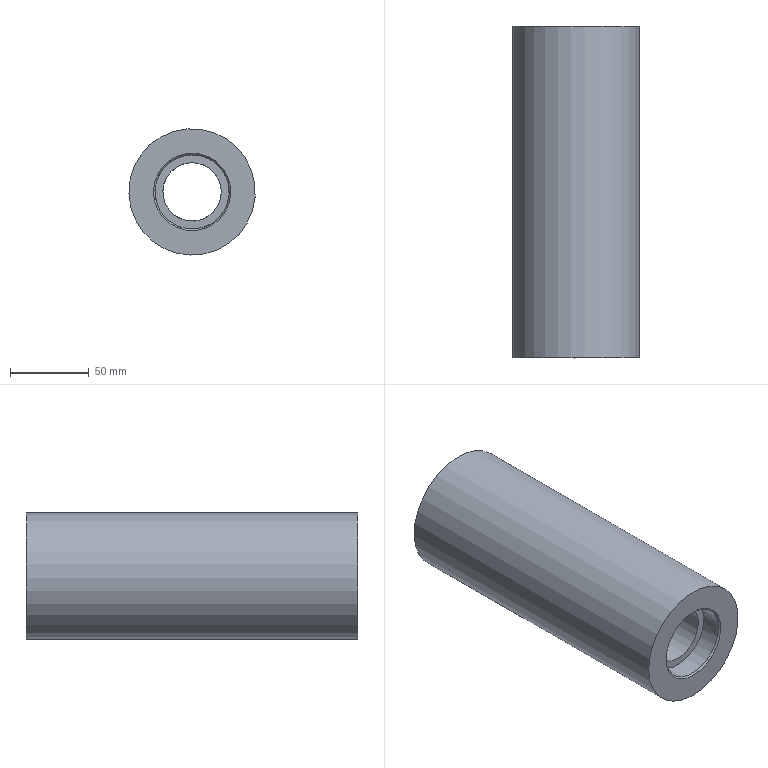Component | NX | 131_ROLLER | 1 solid | 10 faces | box 80 x 210 x 80 mm | volume 811159 mm3 | plane 4 | cylinder 4 | cone 2 | commonest cylinder face diameters 47 x2 80 x1 37 x1
STEP:
#1=CARTESIAN_POINT('',(0.,0.,0.));
#2=DIRECTION('',(0.,0.,1.));
#3=DIRECTION('',(1.,0.,0.));
#4=AXIS2_PLACEMENT_3D('',#1,#2,#3);
#5=CARTESIAN_POINT('',(613.188,-110.,-20.648));
#6=VERTEX_POINT('',#5);
#7=CARTESIAN_POINT('',(600.,-110.,0.));
#8=DIRECTION('',(-0.,1.,-0.));
#9=DIRECTION('',(0.5383,-0.,-0.8428));
#10=AXIS2_PLACEMENT_3D('',#7,#8,#9);
#11=CIRCLE('',#10,24.5);
#12=CARTESIAN_POINT('',(600.,-110.,0.));
#13=DIRECTION('',(0.,-1.,0.));
#14=DIRECTION('',(0.5383,-0.,-0.8428));
#15=AXIS2_PLACEMENT_3D('',#12,#13,#14);
#16=PLANE('',#15);
#17=CARTESIAN_POINT('',(24.5,0.));
#18=CARTESIAN_POINT('',(24.5,-42.435));
#19=CARTESIAN_POINT('',(-12.25,-21.218));
#20=CARTESIAN_POINT('',(-49.,0.));
#21=CARTESIAN_POINT('',(-12.25,21.218));
#22=CARTESIAN_POINT('',(24.5,42.435));
#23=CARTESIAN_POINT('',(24.5,0.));
#24=(BOUNDED_CURVE()B_SPLINE_CURVE(2,(#17,#18,#19,#20,#21,#22,#23),.UNSPECIFIED.,.T.,.F.)B_SPLINE_CURVE_WITH_KNOTS((1,2,2,2,2,1),(-2.094,0.,2.094,4.189,6.283,8.378),.UNSPECIFIED.)CURVE()GEOMETRIC_REPRESENTATION_ITEM()RATIONAL_B_SPLINE_CURVE((1.,0.5,1.,0.5,1.,0.5,1.))REPRESENTATION_ITEM(''));
#25=(GEOMETRIC_REPRESENTATION_CONTEXT(2)PARAMETRIC_REPRESENTATION_CONTEXT()REPRESENTATION_CONTEXT('',''));
#26=DEFINITIONAL_REPRESENTATION('',(#24),#25);
#27=PCURVE('',#16,#26);
#28=CARTESIAN_POINT('',(600.,-110.,0.));
#29=DIRECTION('',(-0.,-1.,0.));
#30=DIRECTION('',(0.5383,-0.,-0.8428));
#31=AXIS2_PLACEMENT_3D('',#28,#29,#30);
#32=CONICAL_SURFACE('',#31,24.5,0.7854);
#33=CARTESIAN_POINT('',(6.283,-0.));
#34=DIRECTION('',(-1.,0.));
#35=VECTOR('',#34,1.);
#36=LINE('',#33,#35);
#37=(GEOMETRIC_REPRESENTATION_CONTEXT(2)PARAMETRIC_REPRESENTATION_CONTEXT()REPRESENTATION_CONTEXT('',''));
#38=DEFINITIONAL_REPRESENTATION('',(#36),#37);
#39=PCURVE('',#32,#38);
#40=SURFACE_CURVE('',#11,(#27,#39),.PCURVE_S1.);
#41=EDGE_CURVE('',#6,#6,#40,.T.);
#42=ORIENTED_EDGE('',*,*,#41,.T.);
#43=EDGE_LOOP('',(#42));
#44=FACE_BOUND('',#43,.T.);
#45=CARTESIAN_POINT('',(633.711,-110.,21.531));
#46=VERTEX_POINT('',#45);
#47=CARTESIAN_POINT('',(600.,-110.,0.));
#48=DIRECTION('',(0.,-1.,0.));
#49=DIRECTION('',(0.8428,0.,0.5383));
#50=AXIS2_PLACEMENT_3D('',#47,#48,#49);
#51=CIRCLE('',#50,40.);
#52=CARTESIAN_POINT('',(-0.,0.));
#53=DIRECTION('',(0.,1.));
#54=AXIS2_PLACEMENT_2D('',#52,#53);
#55=CIRCLE('',#54,40.);
#56=(GEOMETRIC_REPRESENTATION_CONTEXT(2)PARAMETRIC_REPRESENTATION_CONTEXT()REPRESENTATION_CONTEXT('',''));
#57=DEFINITIONAL_REPRESENTATION('',(#55),#56);
#58=PCURVE('',#16,#57);
#59=CARTESIAN_POINT('',(600.,-110.,0.));
#60=DIRECTION('',(-0.,1.,-0.));
#61=DIRECTION('',(-0.5383,0.,0.8428));
#62=AXIS2_PLACEMENT_3D('',#59,#60,#61);
#63=CYLINDRICAL_SURFACE('',#62,40.);
#64=CARTESIAN_POINT('',(7.854,0.));
#65=DIRECTION('',(-1.,0.));
#66=VECTOR('',#65,1.);
#67=LINE('',#64,#66);
#68=(GEOMETRIC_REPRESENTATION_CONTEXT(2)PARAMETRIC_REPRESENTATION_CONTEXT()REPRESENTATION_CONTEXT('',''));
#69=DEFINITIONAL_REPRESENTATION('',(#67),#68);
#70=PCURVE('',#63,#69);
#71=SURFACE_CURVE('',#51,(#58,#70),.PCURVE_S1.);
#72=EDGE_CURVE('',#46,#46,#71,.T.);
#73=ORIENTED_EDGE('',*,*,#72,.T.);
#74=EDGE_LOOP('',(#73));
#75=FACE_BOUND('',#74,.T.);
#76=ADVANCED_FACE('',(#44,#75),#16,.T.);
#77=CARTESIAN_POINT('',(613.188,100.,-20.648));
#78=VERTEX_POINT('',#77);
#79=CARTESIAN_POINT('',(600.,100.,0.));
#80=DIRECTION('',(0.,-1.,0.));
#81=DIRECTION('',(0.5383,-0.,-0.8428));
#82=AXIS2_PLACEMENT_3D('',#79,#80,#81);
#83=CIRCLE('',#82,24.5);
#84=CARTESIAN_POINT('',(600.,100.,0.));
#85=DIRECTION('',(0.,-1.,0.));
#86=DIRECTION('',(0.5383,-0.,-0.8428));
#87=AXIS2_PLACEMENT_3D('',#84,#85,#86);
#88=PLANE('',#87);
#89=CARTESIAN_POINT('',(-0.,0.));
#90=DIRECTION('',(1.,0.));
#91=AXIS2_PLACEMENT_2D('',#89,#90);
#92=CIRCLE('',#91,24.5);
#93=(GEOMETRIC_REPRESENTATION_CONTEXT(2)PARAMETRIC_REPRESENTATION_CONTEXT()REPRESENTATION_CONTEXT('',''));
#94=DEFINITIONAL_REPRESENTATION('',(#92),#93);
#95=PCURVE('',#88,#94);
#96=CARTESIAN_POINT('',(600.,99.,0.));
#97=DIRECTION('',(-0.,1.,0.));
#98=DIRECTION('',(-0.5383,-0.,0.8428));
#99=AXIS2_PLACEMENT_3D('',#96,#97,#98);
#100=CONICAL_SURFACE('',#99,23.5,0.7854);
#101=CARTESIAN_POINT('',(9.425,1.));
#102=DIRECTION('',(-1.,0.));
#103=VECTOR('',#102,1.);
#104=LINE('',#101,#103);
#105=(GEOMETRIC_REPRESENTATION_CONTEXT(2)PARAMETRIC_REPRESENTATION_CONTEXT()REPRESENTATION_CONTEXT('',''));
#106=DEFINITIONAL_REPRESENTATION('',(#104),#105);
#107=PCURVE('',#100,#106);
#108=SURFACE_CURVE('',#83,(#95,#107),.PCURVE_S1.);
#109=EDGE_CURVE('',#78,#78,#108,.T.);
#110=ORIENTED_EDGE('',*,*,#109,.T.);
#111=EDGE_LOOP('',(#110));
#112=FACE_BOUND('',#111,.T.);
#113=CARTESIAN_POINT('',(633.711,100.,21.531));
#114=VERTEX_POINT('',#113);
#115=CARTESIAN_POINT('',(600.,100.,0.));
#116=DIRECTION('',(0.,-1.,0.));
#117=DIRECTION('',(0.8428,0.,0.5383));
#118=AXIS2_PLACEMENT_3D('',#115,#116,#117);
#119=CIRCLE('',#118,40.);
#120=CARTESIAN_POINT('',(-0.,0.));
#121=DIRECTION('',(0.,1.));
#122=AXIS2_PLACEMENT_2D('',#120,#121);
#123=CIRCLE('',#122,40.);
#124=(GEOMETRIC_REPRESENTATION_CONTEXT(2)PARAMETRIC_REPRESENTATION_CONTEXT()REPRESENTATION_CONTEXT('',''));
#125=DEFINITIONAL_REPRESENTATION('',(#123),#124);
#126=PCURVE('',#88,#125);
#127=CARTESIAN_POINT('',(7.854,210.));
#128=DIRECTION('',(-1.,0.));
#129=VECTOR('',#128,1.);
#130=LINE('',#127,#129);
#131=(GEOMETRIC_REPRESENTATION_CONTEXT(2)PARAMETRIC_REPRESENTATION_CONTEXT()REPRESENTATION_CONTEXT('',''));
#132=DEFINITIONAL_REPRESENTATION('',(#130),#131);
#133=PCURVE('',#63,#132);
#134=SURFACE_CURVE('',#119,(#126,#133),.PCURVE_S1.);
#135=EDGE_CURVE('',#114,#114,#134,.T.);
#136=ORIENTED_EDGE('',*,*,#135,.F.);
#137=EDGE_LOOP('',(#136));
#138=FACE_BOUND('',#137,.T.);
#139=ADVANCED_FACE('',(#112,#138),#88,.F.);
#140=ORIENTED_EDGE('',*,*,#72,.F.);
#141=CARTESIAN_POINT('',(633.711,-110.,21.531));
#142=CARTESIAN_POINT('',(633.711,100.,21.531));
#143=B_SPLINE_CURVE_WITH_KNOTS('',1,(#141,#142),.UNSPECIFIED.,.F.,.F.,(2,2),(0.,210.),.PIECEWISE_BEZIER_KNOTS.);
#144=CARTESIAN_POINT('',(7.854,0.));
#145=DIRECTION('',(0.,1.));
#146=VECTOR('',#145,1.);
#147=LINE('',#144,#146);
#148=(GEOMETRIC_REPRESENTATION_CONTEXT(2)PARAMETRIC_REPRESENTATION_CONTEXT()REPRESENTATION_CONTEXT('',''));
#149=DEFINITIONAL_REPRESENTATION('',(#147),#148);
#150=PCURVE('',#63,#149);
#151=CARTESIAN_POINT('',(1.571,0.));
#152=DIRECTION('',(0.,1.));
#153=VECTOR('',#152,1.);
#154=LINE('',#151,#153);
#155=(GEOMETRIC_REPRESENTATION_CONTEXT(2)PARAMETRIC_REPRESENTATION_CONTEXT()REPRESENTATION_CONTEXT('',''));
#156=DEFINITIONAL_REPRESENTATION('',(#154),#155);
#157=PCURVE('',#63,#156);
#158=SEAM_CURVE('',#143,(#150,#157),.PCURVE_S1.);
#159=EDGE_CURVE('',#46,#114,#158,.T.);
#160=ORIENTED_EDGE('',*,*,#159,.T.);
#161=ORIENTED_EDGE('',*,*,#135,.T.);
#162=ORIENTED_EDGE('',*,*,#159,.F.);
#163=EDGE_LOOP('',(#140,#160,#161,#162));
#164=FACE_BOUND('',#163,.T.);
#165=ADVANCED_FACE('',(#164),#63,.T.);
#166=CARTESIAN_POINT('',(619.805,99.,12.649));
#167=VERTEX_POINT('',#166);
#168=CARTESIAN_POINT('',(612.649,99.,-19.805));
#169=VERTEX_POINT('',#168);
#170=CARTESIAN_POINT('',(600.,99.,0.));
#171=DIRECTION('',(-0.,1.,0.));
#172=DIRECTION('',(0.5383,0.,-0.8428));
#173=AXIS2_PLACEMENT_3D('',#170,#171,#172);
#174=CIRCLE('',#173,23.5);
#175=CARTESIAN_POINT('',(600.,86.,0.));
#176=DIRECTION('',(-0.,1.,-0.));
#177=DIRECTION('',(-0.5383,-0.,0.8428));
#178=AXIS2_PLACEMENT_3D('',#175,#176,#177);
#179=CYLINDRICAL_SURFACE('',#178,23.5);
#180=CARTESIAN_POINT('',(-3.142,13.));
#181=DIRECTION('',(1.,0.));
#182=VECTOR('',#181,1.);
#183=LINE('',#180,#182);
#184=(GEOMETRIC_REPRESENTATION_CONTEXT(2)PARAMETRIC_REPRESENTATION_CONTEXT()REPRESENTATION_CONTEXT('',''));
#185=DEFINITIONAL_REPRESENTATION('',(#183),#184);
#186=PCURVE('',#179,#185);
#187=CARTESIAN_POINT('',(3.142,-0.));
#188=DIRECTION('',(1.,0.));
#189=VECTOR('',#188,1.);
#190=LINE('',#187,#189);
#191=(GEOMETRIC_REPRESENTATION_CONTEXT(2)PARAMETRIC_REPRESENTATION_CONTEXT()REPRESENTATION_CONTEXT('',''));
#192=DEFINITIONAL_REPRESENTATION('',(#190),#191);
#193=PCURVE('',#100,#192);
#194=SURFACE_CURVE('',#174,(#186,#193),.PCURVE_S1.);
#195=EDGE_CURVE('',#167,#169,#194,.T.);
#196=ORIENTED_EDGE('',*,*,#195,.F.);
#197=CARTESIAN_POINT('',(619.805,86.,12.649));
#198=VERTEX_POINT('',#197);
#199=CARTESIAN_POINT('',(619.805,86.,12.649));
#200=CARTESIAN_POINT('',(619.805,99.,12.649));
#201=B_SPLINE_CURVE_WITH_KNOTS('',1,(#199,#200),.UNSPECIFIED.,.F.,.F.,(2,2),(0.,13.),.PIECEWISE_BEZIER_KNOTS.);
#202=CARTESIAN_POINT('',(1.571,0.));
#203=DIRECTION('',(0.,1.));
#204=VECTOR('',#203,1.);
#205=LINE('',#202,#204);
#206=(GEOMETRIC_REPRESENTATION_CONTEXT(2)PARAMETRIC_REPRESENTATION_CONTEXT()REPRESENTATION_CONTEXT('',''));
#207=DEFINITIONAL_REPRESENTATION('',(#205),#206);
#208=PCURVE('',#179,#207);
#209=CARTESIAN_POINT('',(7.854,0.));
#210=DIRECTION('',(0.,1.));
#211=VECTOR('',#210,1.);
#212=LINE('',#209,#211);
#213=(GEOMETRIC_REPRESENTATION_CONTEXT(2)PARAMETRIC_REPRESENTATION_CONTEXT()REPRESENTATION_CONTEXT('',''));
#214=DEFINITIONAL_REPRESENTATION('',(#212),#213);
#215=PCURVE('',#179,#214);
#216=SEAM_CURVE('',#201,(#208,#215),.PCURVE_S1.);
#217=EDGE_CURVE('',#198,#167,#216,.T.);
#218=ORIENTED_EDGE('',*,*,#217,.F.);
#219=CARTESIAN_POINT('',(600.,86.,0.));
#220=DIRECTION('',(-0.,-1.,0.));
#221=DIRECTION('',(0.8428,0.,0.5383));
#222=AXIS2_PLACEMENT_3D('',#219,#220,#221);
#223=CIRCLE('',#222,23.5);
#224=CARTESIAN_POINT('',(7.854,0.));
#225=DIRECTION('',(-1.,0.));
#226=VECTOR('',#225,1.);
#227=LINE('',#224,#226);
#228=(GEOMETRIC_REPRESENTATION_CONTEXT(2)PARAMETRIC_REPRESENTATION_CONTEXT()REPRESENTATION_CONTEXT('',''));
#229=DEFINITIONAL_REPRESENTATION('',(#227),#228);
#230=PCURVE('',#179,#229);
#231=CARTESIAN_POINT('',(600.,86.,0.));
#232=DIRECTION('',(-0.,1.,-0.));
#233=DIRECTION('',(-0.5383,0.,0.8428));
#234=AXIS2_PLACEMENT_3D('',#231,#232,#233);
#235=PLANE('',#234);
#236=CARTESIAN_POINT('',(-0.,23.5));
#237=CARTESIAN_POINT('',(40.703,23.5));
#238=CARTESIAN_POINT('',(20.352,-11.75));
#239=CARTESIAN_POINT('',(-0.,-47.));
#240=CARTESIAN_POINT('',(-20.352,-11.75));
#241=CARTESIAN_POINT('',(-40.703,23.5));
#242=CARTESIAN_POINT('',(-0.,23.5));
#243=(BOUNDED_CURVE()B_SPLINE_CURVE(2,(#236,#237,#238,#239,#240,#241,#242),.UNSPECIFIED.,.T.,.F.)B_SPLINE_CURVE_WITH_KNOTS((1,2,2,2,2,1),(-2.094,0.,2.094,4.189,6.283,8.378),.UNSPECIFIED.)CURVE()GEOMETRIC_REPRESENTATION_ITEM()RATIONAL_B_SPLINE_CURVE((1.,0.5,1.,0.5,1.,0.5,1.))REPRESENTATION_ITEM(''));
#244=(GEOMETRIC_REPRESENTATION_CONTEXT(2)PARAMETRIC_REPRESENTATION_CONTEXT()REPRESENTATION_CONTEXT('',''));
#245=DEFINITIONAL_REPRESENTATION('',(#243),#244);
#246=PCURVE('',#235,#245);
#247=SURFACE_CURVE('',#223,(#230,#246),.PCURVE_S1.);
#248=EDGE_CURVE('',#198,#198,#247,.T.);
#249=ORIENTED_EDGE('',*,*,#248,.F.);
#250=ORIENTED_EDGE('',*,*,#217,.T.);
#251=CARTESIAN_POINT('',(600.,99.,0.));
#252=DIRECTION('',(-0.,1.,0.));
#253=DIRECTION('',(0.5383,0.,-0.8428));
#254=AXIS2_PLACEMENT_3D('',#251,#252,#253);
#255=CIRCLE('',#254,23.5);
#256=CARTESIAN_POINT('',(3.142,13.));
#257=DIRECTION('',(1.,0.));
#258=VECTOR('',#257,1.);
#259=LINE('',#256,#258);
#260=(GEOMETRIC_REPRESENTATION_CONTEXT(2)PARAMETRIC_REPRESENTATION_CONTEXT()REPRESENTATION_CONTEXT('',''));
#261=DEFINITIONAL_REPRESENTATION('',(#259),#260);
#262=PCURVE('',#179,#261);
#263=CARTESIAN_POINT('',(3.142,0.));
#264=DIRECTION('',(1.,-0.));
#265=VECTOR('',#264,1.);
#266=LINE('',#263,#265);
#267=(GEOMETRIC_REPRESENTATION_CONTEXT(2)PARAMETRIC_REPRESENTATION_CONTEXT()REPRESENTATION_CONTEXT('',''));
#268=DEFINITIONAL_REPRESENTATION('',(#266),#267);
#269=PCURVE('',#100,#268);
#270=SURFACE_CURVE('',#255,(#262,#269),.PCURVE_S1.);
#271=EDGE_CURVE('',#169,#167,#270,.T.);
#272=ORIENTED_EDGE('',*,*,#271,.F.);
#273=EDGE_LOOP('',(#196,#218,#249,#250,#272));
#274=FACE_BOUND('',#273,.F.);
#275=ADVANCED_FACE('',(#274),#179,.F.);
#276=CARTESIAN_POINT('',(615.591,86.,9.958));
#277=VERTEX_POINT('',#276);
#278=CARTESIAN_POINT('',(590.042,86.,15.591));
#279=VERTEX_POINT('',#278);
#280=CARTESIAN_POINT('',(600.,86.,0.));
#281=DIRECTION('',(0.,1.,-0.));
#282=DIRECTION('',(0.8428,0.,0.5383));
#283=AXIS2_PLACEMENT_3D('',#280,#281,#282);
#284=CIRCLE('',#283,18.5);
#285=CARTESIAN_POINT('',(0.,0.));
#286=DIRECTION('',(0.,1.));
#287=AXIS2_PLACEMENT_2D('',#285,#286);
#288=CIRCLE('',#287,18.5);
#289=(GEOMETRIC_REPRESENTATION_CONTEXT(2)PARAMETRIC_REPRESENTATION_CONTEXT()REPRESENTATION_CONTEXT('',''));
#290=DEFINITIONAL_REPRESENTATION('',(#288),#289);
#291=PCURVE('',#235,#290);
#292=CARTESIAN_POINT('',(600.,-114.,0.));
#293=DIRECTION('',(-0.,1.,-0.));
#294=DIRECTION('',(-0.5383,0.,0.8428));
#295=AXIS2_PLACEMENT_3D('',#292,#293,#294);
#296=CYLINDRICAL_SURFACE('',#295,18.5);
#297=CARTESIAN_POINT('',(1.571,200.));
#298=DIRECTION('',(1.,0.));
#299=VECTOR('',#298,1.);
#300=LINE('',#297,#299);
#301=(GEOMETRIC_REPRESENTATION_CONTEXT(2)PARAMETRIC_REPRESENTATION_CONTEXT()REPRESENTATION_CONTEXT('',''));
#302=DEFINITIONAL_REPRESENTATION('',(#300),#301);
#303=PCURVE('',#296,#302);
#304=SURFACE_CURVE('',#284,(#291,#303),.PCURVE_S1.);
#305=EDGE_CURVE('',#277,#279,#304,.T.);
#306=ORIENTED_EDGE('',*,*,#305,.F.);
#307=CARTESIAN_POINT('',(600.,86.,0.));
#308=DIRECTION('',(0.,1.,-0.));
#309=DIRECTION('',(0.8428,0.,0.5383));
#310=AXIS2_PLACEMENT_3D('',#307,#308,#309);
#311=CIRCLE('',#310,18.5);
#312=CARTESIAN_POINT('',(0.,0.));
#313=DIRECTION('',(0.,1.));
#314=AXIS2_PLACEMENT_2D('',#312,#313);
#315=CIRCLE('',#314,18.5);
#316=(GEOMETRIC_REPRESENTATION_CONTEXT(2)PARAMETRIC_REPRESENTATION_CONTEXT()REPRESENTATION_CONTEXT('',''));
#317=DEFINITIONAL_REPRESENTATION('',(#315),#316);
#318=PCURVE('',#235,#317);
#319=CARTESIAN_POINT('',(-4.712,200.));
#320=DIRECTION('',(1.,0.));
#321=VECTOR('',#320,1.);
#322=LINE('',#319,#321);
#323=(GEOMETRIC_REPRESENTATION_CONTEXT(2)PARAMETRIC_REPRESENTATION_CONTEXT()REPRESENTATION_CONTEXT('',''));
#324=DEFINITIONAL_REPRESENTATION('',(#322),#323);
#325=PCURVE('',#296,#324);
#326=SURFACE_CURVE('',#311,(#318,#325),.PCURVE_S1.);
#327=EDGE_CURVE('',#279,#277,#326,.T.);
#328=ORIENTED_EDGE('',*,*,#327,.F.);
#329=EDGE_LOOP('',(#306,#328));
#330=FACE_BOUND('',#329,.T.);
#331=ORIENTED_EDGE('',*,*,#248,.F.);
#332=EDGE_LOOP('',(#331));
#333=FACE_BOUND('',#332,.T.);
#334=ADVANCED_FACE('',(#330,#333),#235,.T.);
#335=ORIENTED_EDGE('',*,*,#109,.T.);
#336=CARTESIAN_POINT('',(612.649,99.,-19.805));
#337=CARTESIAN_POINT('',(613.188,100.,-20.648));
#338=B_SPLINE_CURVE_WITH_KNOTS('',1,(#336,#337),.UNSPECIFIED.,.F.,.F.,(2,2),(0.,1.414),.PIECEWISE_BEZIER_KNOTS.);
#339=CARTESIAN_POINT('',(3.142,0.));
#340=DIRECTION('',(0.,1.));
#341=VECTOR('',#340,1.);
#342=LINE('',#339,#341);
#343=(GEOMETRIC_REPRESENTATION_CONTEXT(2)PARAMETRIC_REPRESENTATION_CONTEXT()REPRESENTATION_CONTEXT('',''));
#344=DEFINITIONAL_REPRESENTATION('',(#342),#343);
#345=PCURVE('',#100,#344);
#346=CARTESIAN_POINT('',(9.425,0.));
#347=DIRECTION('',(0.,1.));
#348=VECTOR('',#347,1.);
#349=LINE('',#346,#348);
#350=(GEOMETRIC_REPRESENTATION_CONTEXT(2)PARAMETRIC_REPRESENTATION_CONTEXT()REPRESENTATION_CONTEXT('',''));
#351=DEFINITIONAL_REPRESENTATION('',(#349),#350);
#352=PCURVE('',#100,#351);
#353=SEAM_CURVE('',#338,(#345,#352),.PCURVE_S1.);
#354=EDGE_CURVE('',#169,#78,#353,.T.);
#355=ORIENTED_EDGE('',*,*,#354,.F.);
#356=ORIENTED_EDGE('',*,*,#271,.T.);
#357=ORIENTED_EDGE('',*,*,#195,.T.);
#358=ORIENTED_EDGE('',*,*,#354,.T.);
#359=EDGE_LOOP('',(#335,#355,#356,#357,#358));
#360=FACE_BOUND('',#359,.F.);
#361=ADVANCED_FACE('',(#360),#100,.F.);
#362=CARTESIAN_POINT('',(612.649,-109.,-19.805));
#363=VERTEX_POINT('',#362);
#364=CARTESIAN_POINT('',(600.,-109.,0.));
#365=DIRECTION('',(-0.,-1.,0.));
#366=DIRECTION('',(0.5383,-0.,-0.8428));
#367=AXIS2_PLACEMENT_3D('',#364,#365,#366);
#368=CIRCLE('',#367,23.5);
#369=CARTESIAN_POINT('',(600.,-96.,0.));
#370=DIRECTION('',(0.,-1.,0.));
#371=DIRECTION('',(0.5383,0.,-0.8428));
#372=AXIS2_PLACEMENT_3D('',#369,#370,#371);
#373=CYLINDRICAL_SURFACE('',#372,23.5);
#374=CARTESIAN_POINT('',(0.,13.));
#375=DIRECTION('',(1.,0.));
#376=VECTOR('',#375,1.);
#377=LINE('',#374,#376);
#378=(GEOMETRIC_REPRESENTATION_CONTEXT(2)PARAMETRIC_REPRESENTATION_CONTEXT()REPRESENTATION_CONTEXT('',''));
#379=DEFINITIONAL_REPRESENTATION('',(#377),#378);
#380=PCURVE('',#373,#379);
#381=CARTESIAN_POINT('',(0.,-1.));
#382=DIRECTION('',(1.,0.));
#383=VECTOR('',#382,1.);
#384=LINE('',#381,#383);
#385=(GEOMETRIC_REPRESENTATION_CONTEXT(2)PARAMETRIC_REPRESENTATION_CONTEXT()REPRESENTATION_CONTEXT('',''));
#386=DEFINITIONAL_REPRESENTATION('',(#384),#385);
#387=PCURVE('',#32,#386);
#388=SURFACE_CURVE('',#368,(#380,#387),.PCURVE_S1.);
#389=EDGE_CURVE('',#363,#363,#388,.T.);
#390=ORIENTED_EDGE('',*,*,#389,.F.);
#391=CARTESIAN_POINT('',(612.649,-96.,-19.805));
#392=VERTEX_POINT('',#391);
#393=CARTESIAN_POINT('',(612.649,-96.,-19.805));
#394=CARTESIAN_POINT('',(612.649,-109.,-19.805));
#395=B_SPLINE_CURVE_WITH_KNOTS('',1,(#393,#394),.UNSPECIFIED.,.F.,.F.,(2,2),(0.,13.),.PIECEWISE_BEZIER_KNOTS.);
#396=CARTESIAN_POINT('',(0.,0.));
#397=DIRECTION('',(0.,1.));
#398=VECTOR('',#397,1.);
#399=LINE('',#396,#398);
#400=(GEOMETRIC_REPRESENTATION_CONTEXT(2)PARAMETRIC_REPRESENTATION_CONTEXT()REPRESENTATION_CONTEXT('',''));
#401=DEFINITIONAL_REPRESENTATION('',(#399),#400);
#402=PCURVE('',#373,#401);
#403=CARTESIAN_POINT('',(6.283,0.));
#404=DIRECTION('',(0.,1.));
#405=VECTOR('',#404,1.);
#406=LINE('',#403,#405);
#407=(GEOMETRIC_REPRESENTATION_CONTEXT(2)PARAMETRIC_REPRESENTATION_CONTEXT()REPRESENTATION_CONTEXT('',''));
#408=DEFINITIONAL_REPRESENTATION('',(#406),#407);
#409=PCURVE('',#373,#408);
#410=SEAM_CURVE('',#395,(#402,#409),.PCURVE_S1.);
#411=EDGE_CURVE('',#392,#363,#410,.T.);
#412=ORIENTED_EDGE('',*,*,#411,.F.);
#413=CARTESIAN_POINT('',(619.805,-96.,12.649));
#414=VERTEX_POINT('',#413);
#415=CARTESIAN_POINT('',(600.,-96.,0.));
#416=DIRECTION('',(-0.,-1.,0.));
#417=DIRECTION('',(0.8428,0.,0.5383));
#418=AXIS2_PLACEMENT_3D('',#415,#416,#417);
#419=CIRCLE('',#418,23.5);
#420=CARTESIAN_POINT('',(-4.712,0.));
#421=DIRECTION('',(1.,0.));
#422=VECTOR('',#421,1.);
#423=LINE('',#420,#422);
#424=(GEOMETRIC_REPRESENTATION_CONTEXT(2)PARAMETRIC_REPRESENTATION_CONTEXT()REPRESENTATION_CONTEXT('',''));
#425=DEFINITIONAL_REPRESENTATION('',(#423),#424);
#426=PCURVE('',#373,#425);
#427=CARTESIAN_POINT('',(600.,-96.,0.));
#428=DIRECTION('',(-0.,1.,-0.));
#429=DIRECTION('',(-0.5383,0.,0.8428));
#430=AXIS2_PLACEMENT_3D('',#427,#428,#429);
#431=PLANE('',#430);
#432=CARTESIAN_POINT('',(-0.,23.5));
#433=CARTESIAN_POINT('',(40.703,23.5));
#434=CARTESIAN_POINT('',(20.352,-11.75));
#435=CARTESIAN_POINT('',(-0.,-47.));
#436=CARTESIAN_POINT('',(-20.352,-11.75));
#437=CARTESIAN_POINT('',(-40.703,23.5));
#438=CARTESIAN_POINT('',(-0.,23.5));
#439=(BOUNDED_CURVE()B_SPLINE_CURVE(2,(#432,#433,#434,#435,#436,#437,#438),.UNSPECIFIED.,.T.,.F.)B_SPLINE_CURVE_WITH_KNOTS((1,2,2,2,2,1),(-2.094,0.,2.094,4.189,6.283,8.378),.UNSPECIFIED.)CURVE()GEOMETRIC_REPRESENTATION_ITEM()RATIONAL_B_SPLINE_CURVE((1.,0.5,1.,0.5,1.,0.5,1.))REPRESENTATION_ITEM(''));
#440=(GEOMETRIC_REPRESENTATION_CONTEXT(2)PARAMETRIC_REPRESENTATION_CONTEXT()REPRESENTATION_CONTEXT('',''));
#441=DEFINITIONAL_REPRESENTATION('',(#439),#440);
#442=PCURVE('',#431,#441);
#443=SURFACE_CURVE('',#419,(#426,#442),.PCURVE_S1.);
#444=EDGE_CURVE('',#392,#414,#443,.T.);
#445=ORIENTED_EDGE('',*,*,#444,.T.);
#446=CARTESIAN_POINT('',(600.,-96.,0.));
#447=DIRECTION('',(-0.,-1.,0.));
#448=DIRECTION('',(0.8428,0.,0.5383));
#449=AXIS2_PLACEMENT_3D('',#446,#447,#448);
#450=CIRCLE('',#449,23.5);
#451=CARTESIAN_POINT('',(1.571,0.));
#452=DIRECTION('',(1.,0.));
#453=VECTOR('',#452,1.);
#454=LINE('',#451,#453);
#455=(GEOMETRIC_REPRESENTATION_CONTEXT(2)PARAMETRIC_REPRESENTATION_CONTEXT()REPRESENTATION_CONTEXT('',''));
#456=DEFINITIONAL_REPRESENTATION('',(#454),#455);
#457=PCURVE('',#373,#456);
#458=CARTESIAN_POINT('',(-0.,23.5));
#459=CARTESIAN_POINT('',(40.703,23.5));
#460=CARTESIAN_POINT('',(20.352,-11.75));
#461=CARTESIAN_POINT('',(-0.,-47.));
#462=CARTESIAN_POINT('',(-20.352,-11.75));
#463=CARTESIAN_POINT('',(-40.703,23.5));
#464=CARTESIAN_POINT('',(-0.,23.5));
#465=(BOUNDED_CURVE()B_SPLINE_CURVE(2,(#458,#459,#460,#461,#462,#463,#464),.UNSPECIFIED.,.T.,.F.)B_SPLINE_CURVE_WITH_KNOTS((1,2,2,2,2,1),(-2.094,0.,2.094,4.189,6.283,8.378),.UNSPECIFIED.)CURVE()GEOMETRIC_REPRESENTATION_ITEM()RATIONAL_B_SPLINE_CURVE((1.,0.5,1.,0.5,1.,0.5,1.))REPRESENTATION_ITEM(''));
#466=(GEOMETRIC_REPRESENTATION_CONTEXT(2)PARAMETRIC_REPRESENTATION_CONTEXT()REPRESENTATION_CONTEXT('',''));
#467=DEFINITIONAL_REPRESENTATION('',(#465),#466);
#468=PCURVE('',#431,#467);
#469=SURFACE_CURVE('',#450,(#457,#468),.PCURVE_S1.);
#470=EDGE_CURVE('',#414,#392,#469,.T.);
#471=ORIENTED_EDGE('',*,*,#470,.T.);
#472=ORIENTED_EDGE('',*,*,#411,.T.);
#473=EDGE_LOOP('',(#390,#412,#445,#471,#472));
#474=FACE_BOUND('',#473,.F.);
#475=ADVANCED_FACE('',(#474),#373,.F.);
#476=CARTESIAN_POINT('',(590.042,-96.,15.591));
#477=VERTEX_POINT('',#476);
#478=CARTESIAN_POINT('',(600.,-96.,0.));
#479=DIRECTION('',(-0.,1.,-0.));
#480=DIRECTION('',(-0.5383,0.,0.8428));
#481=AXIS2_PLACEMENT_3D('',#478,#479,#480);
#482=CIRCLE('',#481,18.5);
#483=CARTESIAN_POINT('',(-0.,0.));
#484=DIRECTION('',(1.,-0.));
#485=AXIS2_PLACEMENT_2D('',#483,#484);
#486=CIRCLE('',#485,18.5);
#487=(GEOMETRIC_REPRESENTATION_CONTEXT(2)PARAMETRIC_REPRESENTATION_CONTEXT()REPRESENTATION_CONTEXT('',''));
#488=DEFINITIONAL_REPRESENTATION('',(#486),#487);
#489=PCURVE('',#431,#488);
#490=CARTESIAN_POINT('',(0.,18.));
#491=DIRECTION('',(1.,0.));
#492=VECTOR('',#491,1.);
#493=LINE('',#490,#492);
#494=(GEOMETRIC_REPRESENTATION_CONTEXT(2)PARAMETRIC_REPRESENTATION_CONTEXT()REPRESENTATION_CONTEXT('',''));
#495=DEFINITIONAL_REPRESENTATION('',(#493),#494);
#496=PCURVE('',#296,#495);
#497=SURFACE_CURVE('',#482,(#489,#496),.PCURVE_S1.);
#498=EDGE_CURVE('',#477,#477,#497,.T.);
#499=ORIENTED_EDGE('',*,*,#498,.T.);
#500=EDGE_LOOP('',(#499));
#501=FACE_BOUND('',#500,.T.);
#502=ORIENTED_EDGE('',*,*,#470,.T.);
#503=ORIENTED_EDGE('',*,*,#444,.T.);
#504=EDGE_LOOP('',(#502,#503));
#505=FACE_BOUND('',#504,.T.);
#506=ADVANCED_FACE('',(#501,#505),#431,.F.);
#507=ORIENTED_EDGE('',*,*,#389,.T.);
#508=CARTESIAN_POINT('',(612.649,-109.,-19.805));
#509=CARTESIAN_POINT('',(613.188,-110.,-20.648));
#510=B_SPLINE_CURVE_WITH_KNOTS('',1,(#508,#509),.UNSPECIFIED.,.F.,.F.,(2,2),(-1.414,-0.),.PIECEWISE_BEZIER_KNOTS.);
#511=CARTESIAN_POINT('',(6.283,0.));
#512=DIRECTION('',(0.,1.));
#513=VECTOR('',#512,1.);
#514=LINE('',#511,#513);
#515=(GEOMETRIC_REPRESENTATION_CONTEXT(2)PARAMETRIC_REPRESENTATION_CONTEXT()REPRESENTATION_CONTEXT('',''));
#516=DEFINITIONAL_REPRESENTATION('',(#514),#515);
#517=PCURVE('',#32,#516);
#518=CARTESIAN_POINT('',(0.,0.));
#519=DIRECTION('',(0.,1.));
#520=VECTOR('',#519,1.);
#521=LINE('',#518,#520);
#522=(GEOMETRIC_REPRESENTATION_CONTEXT(2)PARAMETRIC_REPRESENTATION_CONTEXT()REPRESENTATION_CONTEXT('',''));
#523=DEFINITIONAL_REPRESENTATION('',(#521),#522);
#524=PCURVE('',#32,#523);
#525=SEAM_CURVE('',#510,(#517,#524),.PCURVE_S1.);
#526=EDGE_CURVE('',#363,#6,#525,.T.);
#527=ORIENTED_EDGE('',*,*,#526,.T.);
#528=ORIENTED_EDGE('',*,*,#41,.T.);
#529=ORIENTED_EDGE('',*,*,#526,.F.);
#530=EDGE_LOOP('',(#507,#527,#528,#529));
#531=FACE_BOUND('',#530,.F.);
#532=ADVANCED_FACE('',(#531),#32,.F.);
#533=ORIENTED_EDGE('',*,*,#327,.F.);
#534=CARTESIAN_POINT('',(590.042,-96.,15.591));
#535=CARTESIAN_POINT('',(590.042,86.,15.591));
#536=B_SPLINE_CURVE_WITH_KNOTS('',1,(#534,#535),.UNSPECIFIED.,.F.,.F.,(2,2),(18.,200.),.PIECEWISE_BEZIER_KNOTS.);
#537=CARTESIAN_POINT('',(0.,0.));
#538=DIRECTION('',(0.,1.));
#539=VECTOR('',#538,1.);
#540=LINE('',#537,#539);
#541=(GEOMETRIC_REPRESENTATION_CONTEXT(2)PARAMETRIC_REPRESENTATION_CONTEXT()REPRESENTATION_CONTEXT('',''));
#542=DEFINITIONAL_REPRESENTATION('',(#540),#541);
#543=PCURVE('',#296,#542);
#544=CARTESIAN_POINT('',(6.283,0.));
#545=DIRECTION('',(0.,1.));
#546=VECTOR('',#545,1.);
#547=LINE('',#544,#546);
#548=(GEOMETRIC_REPRESENTATION_CONTEXT(2)PARAMETRIC_REPRESENTATION_CONTEXT()REPRESENTATION_CONTEXT('',''));
#549=DEFINITIONAL_REPRESENTATION('',(#547),#548);
#550=PCURVE('',#296,#549);
#551=SEAM_CURVE('',#536,(#543,#550),.PCURVE_S1.);
#552=EDGE_CURVE('',#477,#279,#551,.T.);
#553=ORIENTED_EDGE('',*,*,#552,.F.);
#554=ORIENTED_EDGE('',*,*,#498,.T.);
#555=ORIENTED_EDGE('',*,*,#552,.T.);
#556=ORIENTED_EDGE('',*,*,#305,.F.);
#557=EDGE_LOOP('',(#533,#553,#554,#555,#556));
#558=FACE_BOUND('',#557,.F.);
#559=ADVANCED_FACE('',(#558),#296,.F.);
#560=CLOSED_SHELL('',(#76,#139,#165,#275,#334,#361,#475,#506,#532,#559));
#561=MANIFOLD_SOLID_BREP('',#560);
#562=(LENGTH_UNIT()NAMED_UNIT(*)SI_UNIT(.MILLI.,.METRE.));
#563=UNCERTAINTY_MEASURE_WITH_UNIT(LENGTH_MEASURE(0.000005),#562,'','');
#564=(NAMED_UNIT(*)PLANE_ANGLE_UNIT()SI_UNIT($,.RADIAN.));
#565=(NAMED_UNIT(*)SI_UNIT($,.STERADIAN.)SOLID_ANGLE_UNIT());
#566=(GEOMETRIC_REPRESENTATION_CONTEXT(3)GLOBAL_UNCERTAINTY_ASSIGNED_CONTEXT((#563))GLOBAL_UNIT_ASSIGNED_CONTEXT((#562,#564,#565))REPRESENTATION_CONTEXT('',''));
#567=ADVANCED_BREP_SHAPE_REPRESENTATION('',(#4,#561),#566);